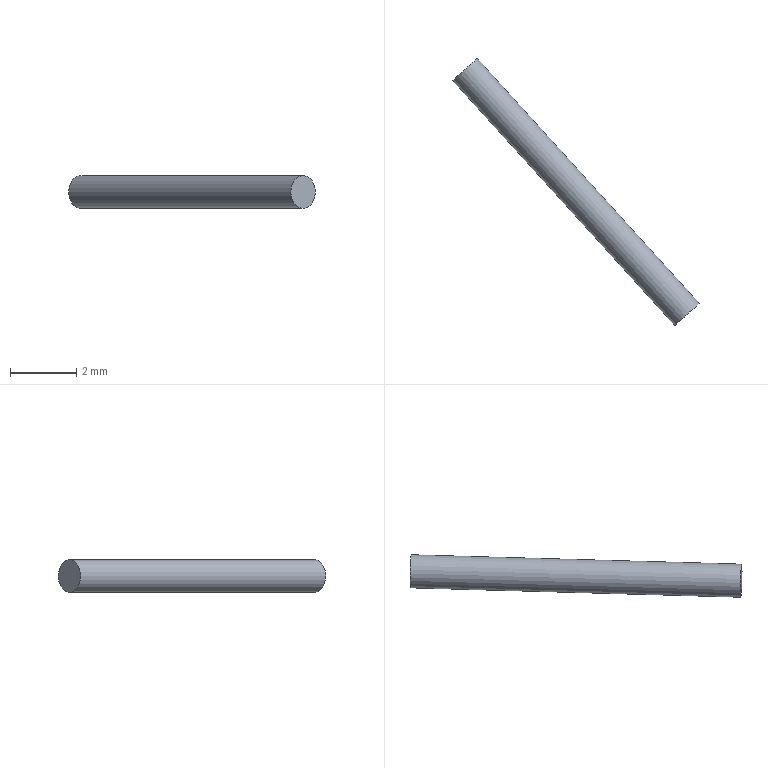Component | NX | CRANK_ROCKER_3_FIXED | 1 solid | 3 faces | box 7.46 x 8.08 x 1 mm | volume 8 mm3 | plane 2 | cylinder 1 | commonest cylinder face diameters 1 x1
STEP:
#1=CARTESIAN_POINT('',(0.,0.,0.));
#2=DIRECTION('',(0.,0.,1.));
#3=DIRECTION('',(1.,0.,0.));
#4=AXIS2_PLACEMENT_3D('',#1,#2,#3);
#5=CARTESIAN_POINT('',(32.847,-19.546,-7.373));
#6=VERTEX_POINT('',#5);
#7=CARTESIAN_POINT('',(33.207,-19.22,-7.49));
#8=DIRECTION('',(-0.6716,0.7409,0.));
#9=DIRECTION('',(-0.72,-0.6527,0.2359));
#10=AXIS2_PLACEMENT_3D('',#7,#8,#9);
#11=CIRCLE('',#10,0.5);
#12=CARTESIAN_POINT('',(33.207,-19.22,-7.49));
#13=DIRECTION('',(-0.6716,0.7409,0.));
#14=DIRECTION('',(-0.72,-0.6527,0.2359));
#15=AXIS2_PLACEMENT_3D('',#12,#13,#14);
#16=CYLINDRICAL_SURFACE('',#15,0.5);
#17=CARTESIAN_POINT('',(0.,0.));
#18=DIRECTION('',(1.,0.));
#19=VECTOR('',#18,1.);
#20=LINE('',#17,#19);
#21=(GEOMETRIC_REPRESENTATION_CONTEXT(2)PARAMETRIC_REPRESENTATION_CONTEXT()REPRESENTATION_CONTEXT('',''));
#22=DEFINITIONAL_REPRESENTATION('',(#20),#21);
#23=PCURVE('',#16,#22);
#24=CARTESIAN_POINT('',(33.207,-19.22,-7.49));
#25=DIRECTION('',(-0.6716,0.7409,0.));
#26=DIRECTION('',(-0.72,-0.6527,0.2359));
#27=AXIS2_PLACEMENT_3D('',#24,#25,#26);
#28=PLANE('',#27);
#29=CARTESIAN_POINT('',(0.,0.));
#30=DIRECTION('',(1.,0.));
#31=AXIS2_PLACEMENT_2D('',#29,#30);
#32=CIRCLE('',#31,0.5);
#33=(GEOMETRIC_REPRESENTATION_CONTEXT(2)PARAMETRIC_REPRESENTATION_CONTEXT()REPRESENTATION_CONTEXT('',''));
#34=DEFINITIONAL_REPRESENTATION('',(#32),#33);
#35=PCURVE('',#28,#34);
#36=SURFACE_CURVE('',#11,(#23,#35),.PCURVE_S1.);
#37=EDGE_CURVE('',#6,#6,#36,.T.);
#38=ORIENTED_EDGE('',*,*,#37,.T.);
#39=CARTESIAN_POINT('',(26.131,-12.137,-7.373));
#40=VERTEX_POINT('',#39);
#41=CARTESIAN_POINT('',(32.847,-19.546,-7.373));
#42=CARTESIAN_POINT('',(26.131,-12.137,-7.373));
#43=B_SPLINE_CURVE_WITH_KNOTS('',1,(#41,#42),.UNSPECIFIED.,.F.,.F.,(2,2),(0.,10.),.PIECEWISE_BEZIER_KNOTS.);
#44=CARTESIAN_POINT('',(6.283,0.));
#45=DIRECTION('',(0.,1.));
#46=VECTOR('',#45,1.);
#47=LINE('',#44,#46);
#48=(GEOMETRIC_REPRESENTATION_CONTEXT(2)PARAMETRIC_REPRESENTATION_CONTEXT()REPRESENTATION_CONTEXT('',''));
#49=DEFINITIONAL_REPRESENTATION('',(#47),#48);
#50=PCURVE('',#16,#49);
#51=CARTESIAN_POINT('',(0.,0.));
#52=DIRECTION('',(0.,1.));
#53=VECTOR('',#52,1.);
#54=LINE('',#51,#53);
#55=(GEOMETRIC_REPRESENTATION_CONTEXT(2)PARAMETRIC_REPRESENTATION_CONTEXT()REPRESENTATION_CONTEXT('',''));
#56=DEFINITIONAL_REPRESENTATION('',(#54),#55);
#57=PCURVE('',#16,#56);
#58=SEAM_CURVE('',#43,(#50,#57),.PCURVE_S1.);
#59=EDGE_CURVE('',#6,#40,#58,.T.);
#60=ORIENTED_EDGE('',*,*,#59,.T.);
#61=CARTESIAN_POINT('',(26.491,-11.811,-7.49));
#62=DIRECTION('',(-0.6716,0.7409,0.));
#63=DIRECTION('',(-0.72,-0.6527,0.2359));
#64=AXIS2_PLACEMENT_3D('',#61,#62,#63);
#65=CIRCLE('',#64,0.5);
#66=CARTESIAN_POINT('',(0.,10.));
#67=DIRECTION('',(1.,0.));
#68=VECTOR('',#67,1.);
#69=LINE('',#66,#68);
#70=(GEOMETRIC_REPRESENTATION_CONTEXT(2)PARAMETRIC_REPRESENTATION_CONTEXT()REPRESENTATION_CONTEXT('',''));
#71=DEFINITIONAL_REPRESENTATION('',(#69),#70);
#72=PCURVE('',#16,#71);
#73=CARTESIAN_POINT('',(26.491,-11.811,-7.49));
#74=DIRECTION('',(-0.6716,0.7409,0.));
#75=DIRECTION('',(-0.72,-0.6527,0.2359));
#76=AXIS2_PLACEMENT_3D('',#73,#74,#75);
#77=PLANE('',#76);
#78=CARTESIAN_POINT('',(0.,0.));
#79=DIRECTION('',(1.,-0.));
#80=AXIS2_PLACEMENT_2D('',#78,#79);
#81=CIRCLE('',#80,0.5);
#82=(GEOMETRIC_REPRESENTATION_CONTEXT(2)PARAMETRIC_REPRESENTATION_CONTEXT()REPRESENTATION_CONTEXT('',''));
#83=DEFINITIONAL_REPRESENTATION('',(#81),#82);
#84=PCURVE('',#77,#83);
#85=SURFACE_CURVE('',#65,(#72,#84),.PCURVE_S1.);
#86=EDGE_CURVE('',#40,#40,#85,.T.);
#87=ORIENTED_EDGE('',*,*,#86,.F.);
#88=ORIENTED_EDGE('',*,*,#59,.F.);
#89=EDGE_LOOP('',(#38,#60,#87,#88));
#90=FACE_BOUND('',#89,.T.);
#91=ADVANCED_FACE('',(#90),#16,.T.);
#92=ORIENTED_EDGE('',*,*,#37,.F.);
#93=EDGE_LOOP('',(#92));
#94=FACE_BOUND('',#93,.T.);
#95=ADVANCED_FACE('',(#94),#28,.F.);
#96=ORIENTED_EDGE('',*,*,#86,.T.);
#97=EDGE_LOOP('',(#96));
#98=FACE_BOUND('',#97,.T.);
#99=ADVANCED_FACE('',(#98),#77,.T.);
#100=CLOSED_SHELL('',(#91,#95,#99));
#101=MANIFOLD_SOLID_BREP('',#100);
#102=(LENGTH_UNIT()NAMED_UNIT(*)SI_UNIT(.MILLI.,.METRE.));
#103=UNCERTAINTY_MEASURE_WITH_UNIT(LENGTH_MEASURE(0.00001),#102,'','');
#104=(NAMED_UNIT(*)PLANE_ANGLE_UNIT()SI_UNIT($,.RADIAN.));
#105=(NAMED_UNIT(*)SI_UNIT($,.STERADIAN.)SOLID_ANGLE_UNIT());
#106=(GEOMETRIC_REPRESENTATION_CONTEXT(3)GLOBAL_UNCERTAINTY_ASSIGNED_CONTEXT((#103))GLOBAL_UNIT_ASSIGNED_CONTEXT((#102,#104,#105))REPRESENTATION_CONTEXT('',''));
#107=ADVANCED_BREP_SHAPE_REPRESENTATION('',(#4,#101),#106);